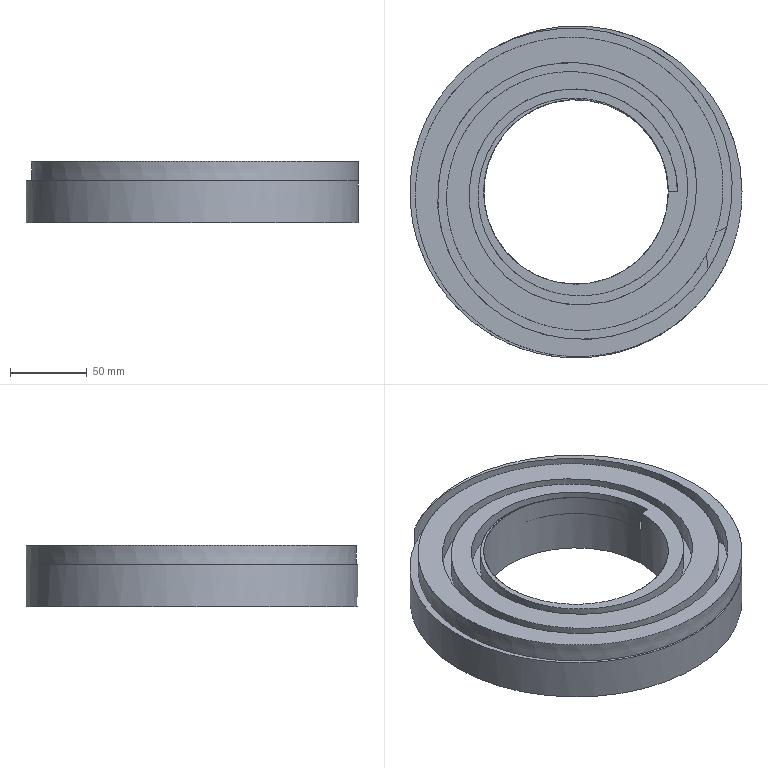Component | NX | SCREW_PLATE | 1 solid | 24 faces | volume 908476 mm3 | cylinder 10 | cone 8 | plane 4 | spline 1 | other 1 | commonest cylinder face diameters 5 x8 216 x1 120 x1